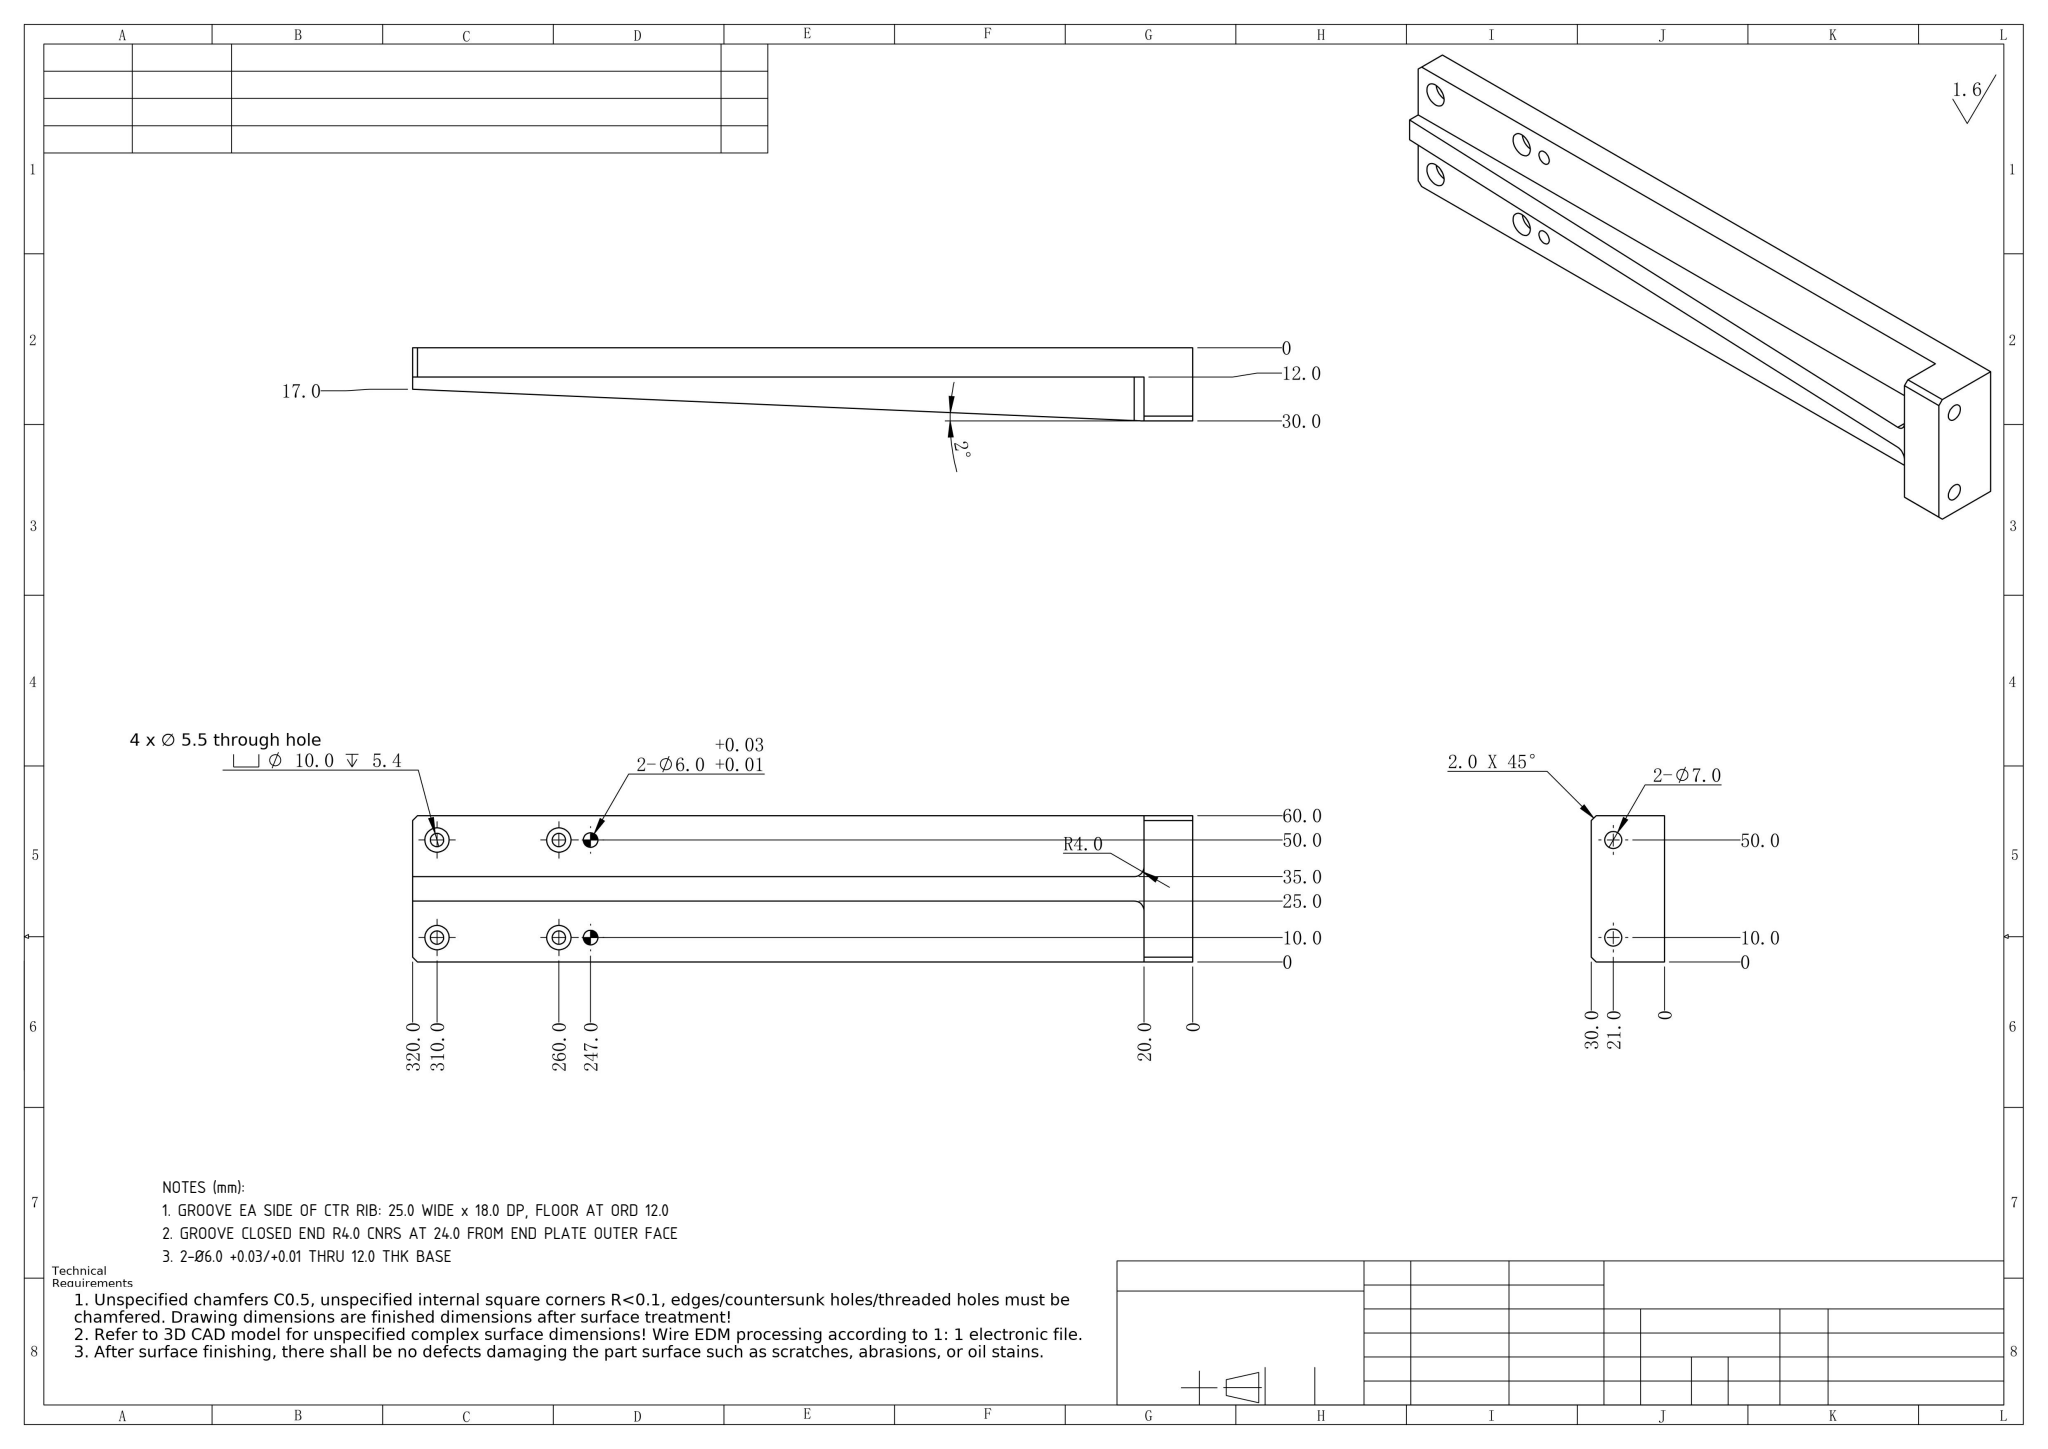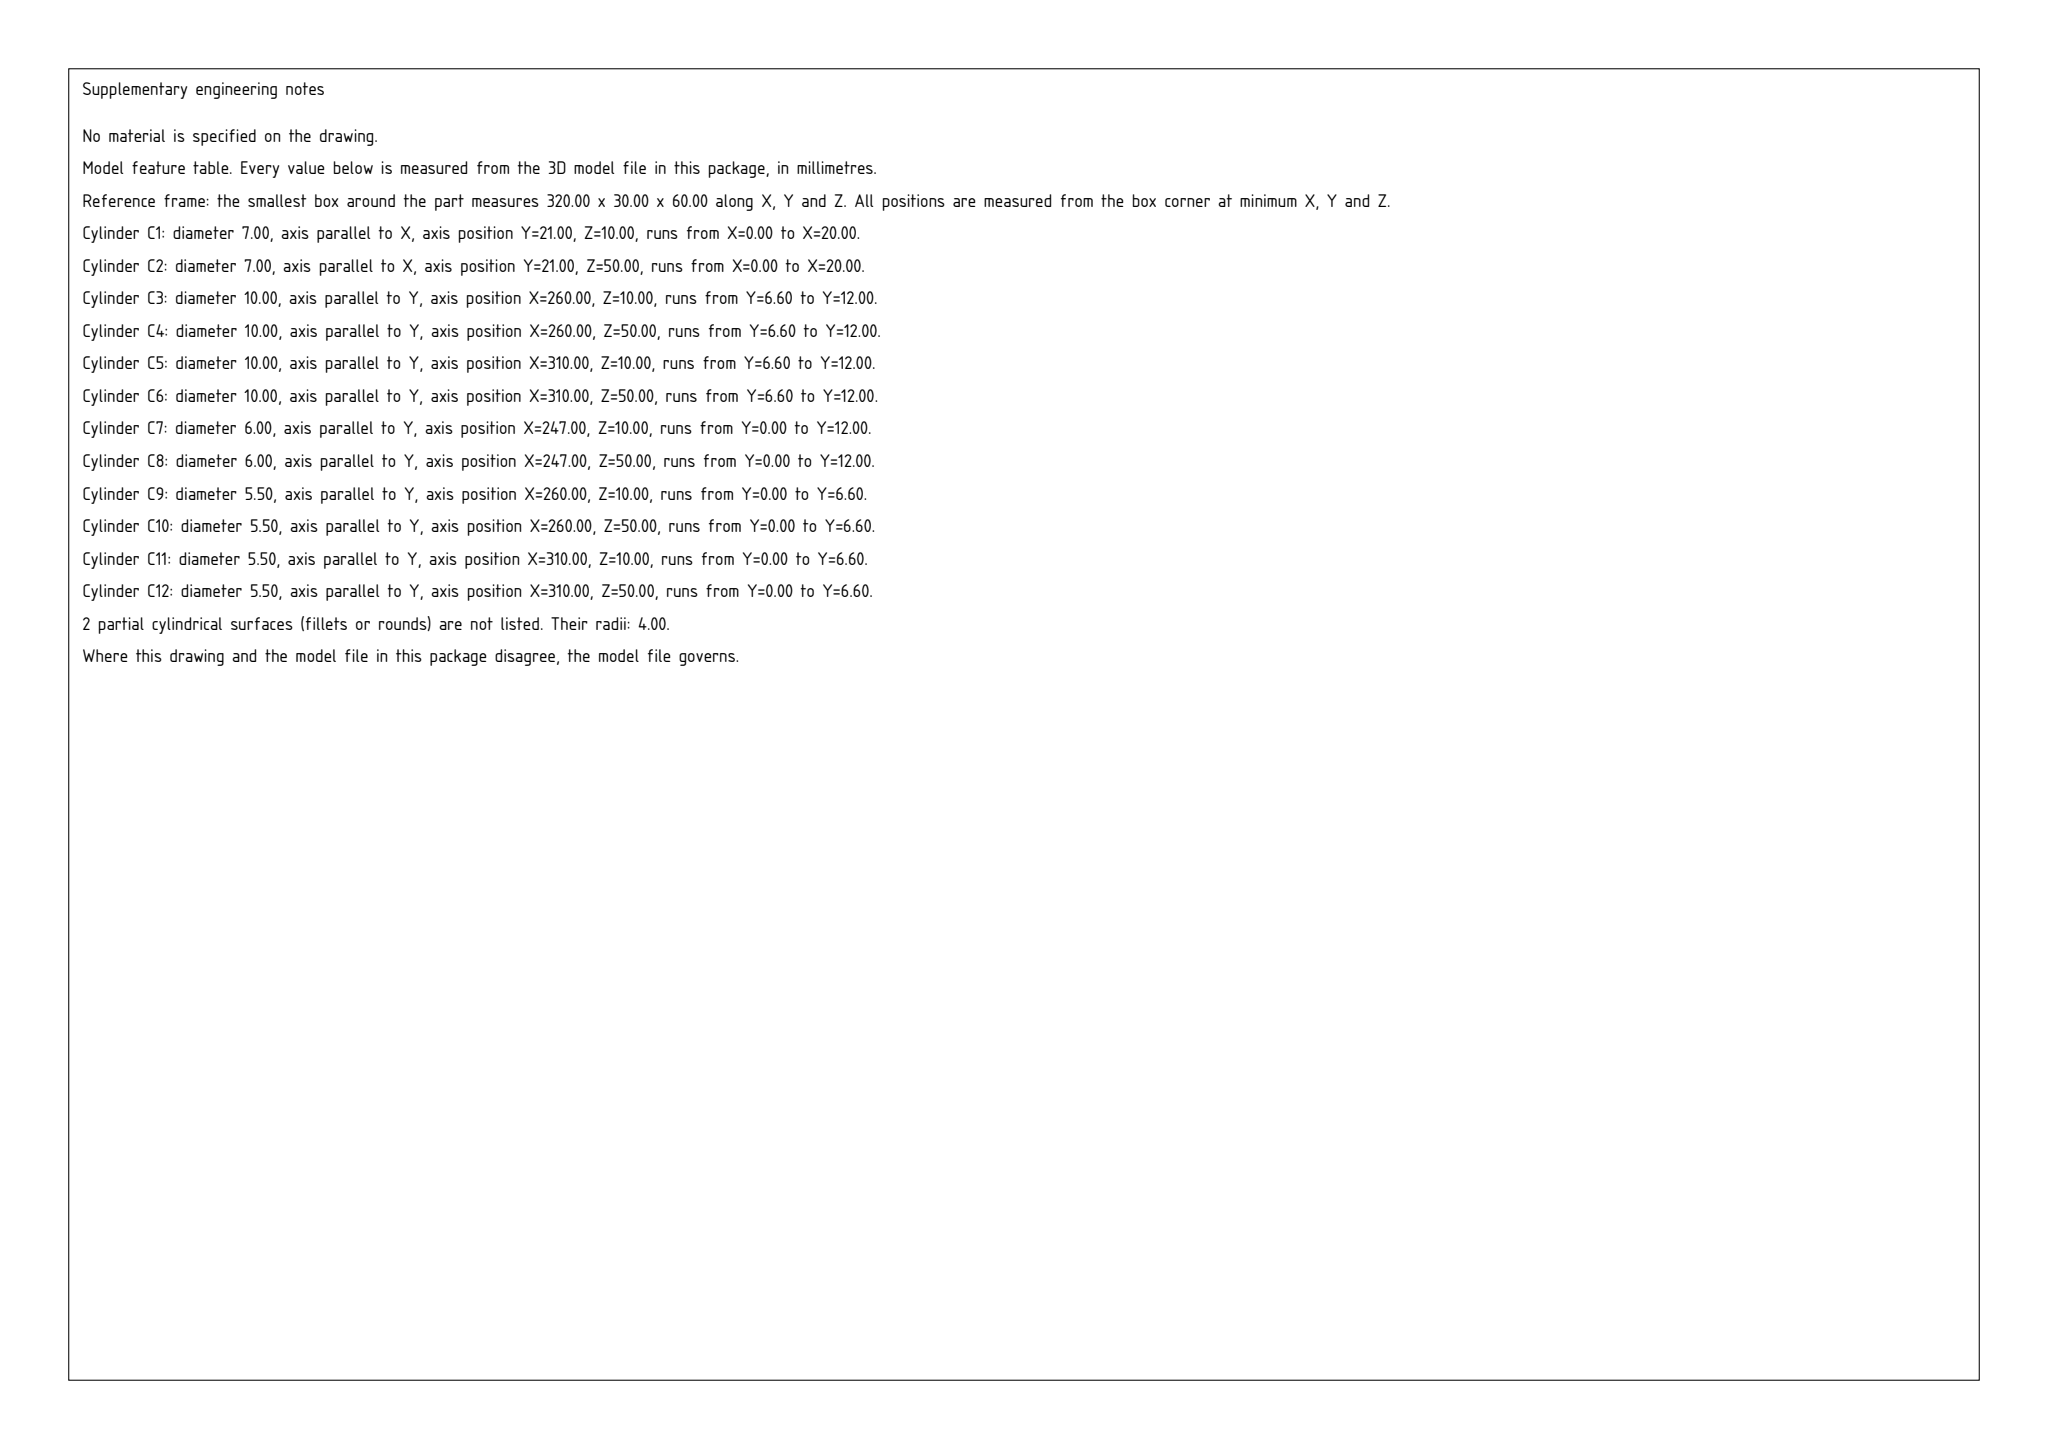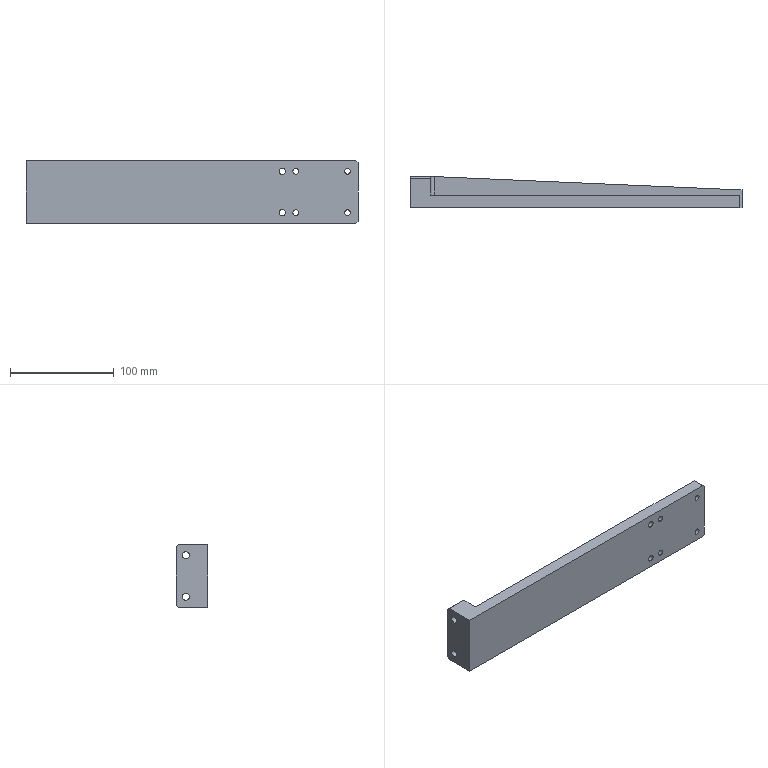Part | SolidWorks | mm | 1 solid | 47 faces | box 320 x 30 x 60 mm | volume 281954 mm3 | cylinder 26 | plane 21 | commonest cylinder face diameters 10 x8 5.5 x8 6 x4 7 x4 8 x2
Drawing notes:
GROOVE EA SIDE OF CTR RIB: 25.0 WIDE x 18.0 DP, FLOOR AT ORD 12.0 | from the solid: z-planes 25.0/35.0 = 10 wide CL rib walls; y-plane 12.0 = groove floors; Ø8 y-cyls len 18.0 (y12->y30)
GROOVE CLOSED END R4.0 CNRS AT 24.0 FROM END PLATE OUTER FACE | from the solid: Ø8.0 y-axis cyls at x=24.0, z=21.0 & 39.0 tangent to rib walls z=25/35; end plate faces x=0 and x=20.0
2-Ø6.0 +0.03/+0.01 THRU 12.0 THK BASE | from the solid: Ø6.0 y-axis cylinders at x=247.0, z=10.0 & 50.0, length 12.0 = base thk (y-planes 0 and 12.0)